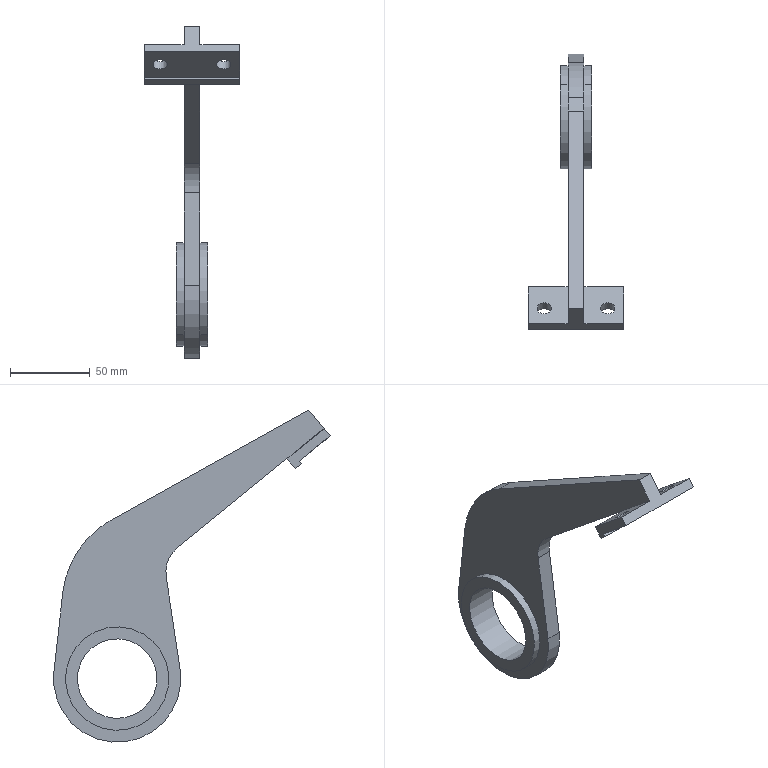Component | SolidWorks | OT-0100-003(SwingRod)-1 | 1 solid | 31 faces | box 60 x 173.77 x 208.81 mm | volume 126646 mm3 | plane 17 | cylinder 14 | commonest cylinder face diameters 9 x4 65 x4 50 x2 120 x2 40 x1 80 x1 | material Plain Carbon Steel
build123d program:
from build123d import *

# Parameters (mm, degrees)
BOSS_EXTRUDE1_DEPTH = 5
SKETCH2_R           = 32.5
BOSS_EXTRUDE2_DEPTH = 10
SKETCH3_R           = 25
CUT_EXTRUDE1_DEPTH  = 20
SKETCH4_W           = 60
SKETCH4_H           = 30
BOSS_EXTRUDE3_DEPTH = 8
CUT_EXTRUDE2_REACH  = 225.825
SKETCH5_W           = 2
SKETCH5_H           = 25
CUT_EXTRUDE3_REACH  = 219.486
SKETCH6_R           = 4.5


with BuildPart() as part:
    # Sketch1 → Boss-Extrude1 (new, symmetric)
    with BuildSketch(Plane(origin=(0, 0, 0), x_dir=(0, 0, -1), z_dir=(1, 0, 0))):
        with BuildLine():
            Line((-63.411, -7.471), (-28.535, 28.031))
            ThreePointArc((-28.535, 28.031), (31.516, 24.632), (20.308, -34.462))
            Line((20.308, -34.462), (-30.154, -64.198))
            ThreePointArc((-30.154, -64.198), (-37.365, -71.506), (-40, -81.429))
            Line((-40, -81.429), (-40, -200))
            Line((-40, -200), (-55, -200))
            Line((-55, -200), (-79.697, -59.937))
            ThreePointArc((-79.697, -59.937), (-77.911, -31.731), (-63.411, -7.471))
        make_face()
    extrude(amount=BOSS_EXTRUDE1_DEPTH, both=True)

    # Sketch2 → Boss-Extrude2 (add, symmetric)
    with BuildSketch(Plane(origin=(0, 0, 0), x_dir=(0, 0, -1), z_dir=(1, 0, 0))):
        with Locations(Location((0, 0, 0), (0, 0, 180))):
            Circle(SKETCH2_R)
    extrude(amount=BOSS_EXTRUDE2_DEPTH, both=True)

    # Sketch3 → Cut-Extrude1 (cut)
    with BuildSketch(Plane(origin=(10, 0, 0), x_dir=(0, 0, -1), z_dir=(1, 0, 0))):
        Circle(SKETCH3_R)
    extrude(amount=-CUT_EXTRUDE1_DEPTH, mode=Mode.SUBTRACT)

    # Sketch4 → Boss-Extrude3 (add)
    with BuildSketch(Plane(origin=(0, 0, 40), x_dir=(-1, 0, 0), z_dir=(0, 0, -1))):
        with Locations((0, -185)):
            Rectangle(SKETCH4_W, SKETCH4_H)
    extrude(amount=BOSS_EXTRUDE3_DEPTH)

    # Sketch5 → Cut-Extrude2 (cut, up to next)
    with BuildSketch(Plane(origin=(30, 0, 0), x_dir=(0, 0, -1), z_dir=(1, 0, 0)), mode=Mode.PRIVATE) as cut_extrude2_sk1:
        with Locations((-33, -187.5)):
            Rectangle(SKETCH5_W, SKETCH5_H)
    cut_extrude2_tool1 = extrude(cut_extrude2_sk1.sketch, amount=-CUT_EXTRUDE2_REACH, mode=Mode.PRIVATE) & part.part
    add(cut_extrude2_tool1.solids().sort_by_distance((30, -187.5, 33))[0], mode=Mode.SUBTRACT)

    # Sketch6 → Cut-Extrude3 (cut, up to next)
    with BuildSketch(Plane.XY.offset(40), mode=Mode.PRIVATE) as cut_extrude3_sk1:
        with Locations((20, -187.5)):
            Circle(SKETCH6_R)
    cut_extrude3_tool1 = extrude(cut_extrude3_sk1.sketch, amount=-CUT_EXTRUDE3_REACH, mode=Mode.PRIVATE) & part.part
    # Sketch6 → Cut-Extrude3 (cut, up to next)
    with BuildSketch(Plane.XY.offset(40), mode=Mode.PRIVATE) as cut_extrude3_sk2:
        with Locations((-20, -187.5)):
            Circle(SKETCH6_R)
    cut_extrude3_tool2 = extrude(cut_extrude3_sk2.sketch, amount=-CUT_EXTRUDE3_REACH, mode=Mode.PRIVATE) & part.part
    add(cut_extrude3_tool1.solids().sort_by_distance((20, -187.5, 40))[0], mode=Mode.SUBTRACT)
    add(cut_extrude3_tool2.solids().sort_by_distance((-20, -187.5, 40))[0], mode=Mode.SUBTRACT)


solid = part.part

# Placed as in the assembly
solid = solid.moved(Location((-20, 35, 0), (-39.097, 0, 0)))
STEP:
#1=COLOUR_RGB('',0.7922,0.8196,0.9333);
#2=FILL_AREA_STYLE_COLOUR('',#1);
#3=FILL_AREA_STYLE('',(#2));
#4=SURFACE_STYLE_FILL_AREA(#3);
#5=SURFACE_SIDE_STYLE('',(#4));
#6=SURFACE_STYLE_USAGE(.BOTH.,#5);
#7=PRESENTATION_STYLE_ASSIGNMENT((#6));
#8=CARTESIAN_POINT('',(-1.398,-3.507,5.694));
#9=VERTEX_POINT('',#8);
#10=CARTESIAN_POINT('',(-1.752,-3.507,5.694));
#11=VERTEX_POINT('',#10);
#12=CARTESIAN_POINT('',(-1.575,-3.507,5.694));
#13=DIRECTION('',(0.,-0.6306,-0.7761));
#14=DIRECTION('',(1.,0.,0.));
#15=AXIS2_PLACEMENT_3D('',#12,#13,#14);
#16=CIRCLE('',#15,0.1772);
#17=EDGE_CURVE('',#9,#11,#16,.T.);
#18=ORIENTED_EDGE('',*,*,#17,.T.);
#19=CARTESIAN_POINT('',(-1.752,-3.358,5.877));
#20=VERTEX_POINT('',#19);
#21=CARTESIAN_POINT('',(-1.752,-5.344,3.433));
#22=DIRECTION('',(-0.,0.6306,0.7761));
#23=VECTOR('',#22,39.37);
#24=LINE('',#21,#23);
#25=EDGE_CURVE('',#11,#20,#24,.T.);
#26=ORIENTED_EDGE('',*,*,#25,.T.);
#27=CARTESIAN_POINT('',(-1.398,-3.358,5.877));
#28=VERTEX_POINT('',#27);
#29=CARTESIAN_POINT('',(-1.575,-3.358,5.877));
#30=DIRECTION('',(-0.,0.6306,0.7761));
#31=DIRECTION('',(-1.,0.,0.));
#32=AXIS2_PLACEMENT_3D('',#29,#30,#31);
#33=CIRCLE('',#32,0.1772);
#34=EDGE_CURVE('',#20,#28,#33,.T.);
#35=ORIENTED_EDGE('',*,*,#34,.T.);
#36=CARTESIAN_POINT('',(-1.398,-5.344,3.433));
#37=DIRECTION('',(-0.,0.6306,0.7761));
#38=VECTOR('',#37,39.37);
#39=LINE('',#36,#38);
#40=EDGE_CURVE('',#9,#28,#39,.T.);
#41=ORIENTED_EDGE('',*,*,#40,.F.);
#42=EDGE_LOOP('',(#18,#26,#35,#41));
#43=FACE_OUTER_BOUND('',#42,.T.);
#44=CARTESIAN_POINT('',(-1.575,-5.344,3.433));
#45=DIRECTION('',(-0.,0.6306,0.7761));
#46=DIRECTION('',(1.,0.,0.));
#47=AXIS2_PLACEMENT_3D('',#44,#45,#46);
#48=CYLINDRICAL_SURFACE('',#47,0.1772);
#49=ADVANCED_FACE('',(#43),#48,.F.);
#50=CARTESIAN_POINT('',(0.1772,-3.507,5.694));
#51=VERTEX_POINT('',#50);
#52=CARTESIAN_POINT('',(-0.1772,-3.507,5.694));
#53=VERTEX_POINT('',#52);
#54=CARTESIAN_POINT('',(0.,-3.507,5.694));
#55=DIRECTION('',(0.,-0.6306,-0.7761));
#56=DIRECTION('',(1.,0.,0.));
#57=AXIS2_PLACEMENT_3D('',#54,#55,#56);
#58=CIRCLE('',#57,0.1772);
#59=EDGE_CURVE('',#51,#53,#58,.T.);
#60=ORIENTED_EDGE('',*,*,#59,.T.);
#61=CARTESIAN_POINT('',(-0.1772,-3.358,5.877));
#62=VERTEX_POINT('',#61);
#63=CARTESIAN_POINT('',(-0.1772,-5.344,3.433));
#64=DIRECTION('',(-0.,0.6306,0.7761));
#65=VECTOR('',#64,39.37);
#66=LINE('',#63,#65);
#67=EDGE_CURVE('',#53,#62,#66,.T.);
#68=ORIENTED_EDGE('',*,*,#67,.T.);
#69=CARTESIAN_POINT('',(0.1772,-3.358,5.877));
#70=VERTEX_POINT('',#69);
#71=CARTESIAN_POINT('',(0.,-3.358,5.877));
#72=DIRECTION('',(-0.,0.6306,0.7761));
#73=DIRECTION('',(1.,0.,0.));
#74=AXIS2_PLACEMENT_3D('',#71,#72,#73);
#75=CIRCLE('',#74,0.1772);
#76=EDGE_CURVE('',#62,#70,#75,.T.);
#77=ORIENTED_EDGE('',*,*,#76,.T.);
#78=CARTESIAN_POINT('',(0.1772,-5.344,3.433));
#79=DIRECTION('',(-0.,0.6306,0.7761));
#80=VECTOR('',#79,39.37);
#81=LINE('',#78,#80);
#82=EDGE_CURVE('',#51,#70,#81,.T.);
#83=ORIENTED_EDGE('',*,*,#82,.F.);
#84=EDGE_LOOP('',(#60,#68,#77,#83));
#85=FACE_OUTER_BOUND('',#84,.T.);
#86=CARTESIAN_POINT('',(0.,-5.344,3.433));
#87=DIRECTION('',(-0.,0.6306,0.7761));
#88=DIRECTION('',(1.,0.,0.));
#89=AXIS2_PLACEMENT_3D('',#86,#87,#88);
#90=CYLINDRICAL_SURFACE('',#89,0.1772);
#91=ADVANCED_FACE('',(#85),#90,.F.);
#92=CARTESIAN_POINT('',(-1.181,1.999,0.7639));
#93=VERTEX_POINT('',#92);
#94=CARTESIAN_POINT('',(-1.181,0.7573,-0.7639));
#95=VERTEX_POINT('',#94);
#96=CARTESIAN_POINT('',(-1.181,1.378,0.));
#97=DIRECTION('',(1.,0.,-0.));
#98=DIRECTION('',(0.,-0.6306,-0.7761));
#99=AXIS2_PLACEMENT_3D('',#96,#97,#98);
#100=CIRCLE('',#99,0.9843);
#101=EDGE_CURVE('',#93,#95,#100,.T.);
#102=ORIENTED_EDGE('',*,*,#101,.F.);
#103=CARTESIAN_POINT('',(-0.3937,1.999,0.7639));
#104=VERTEX_POINT('',#103);
#105=CARTESIAN_POINT('',(-1.181,1.999,0.7639));
#106=DIRECTION('',(1.,0.,-0.));
#107=VECTOR('',#106,39.37);
#108=LINE('',#105,#107);
#109=EDGE_CURVE('',#93,#104,#108,.T.);
#110=ORIENTED_EDGE('',*,*,#109,.T.);
#111=CARTESIAN_POINT('',(-0.3937,0.7573,-0.7639));
#112=VERTEX_POINT('',#111);
#113=CARTESIAN_POINT('',(-0.3937,1.378,0.));
#114=DIRECTION('',(1.,0.,-0.));
#115=DIRECTION('',(0.,-0.6306,-0.7761));
#116=AXIS2_PLACEMENT_3D('',#113,#114,#115);
#117=CIRCLE('',#116,0.9843);
#118=EDGE_CURVE('',#104,#112,#117,.T.);
#119=ORIENTED_EDGE('',*,*,#118,.T.);
#120=CARTESIAN_POINT('',(-1.181,0.7573,-0.7639));
#121=DIRECTION('',(1.,0.,-0.));
#122=VECTOR('',#121,39.37);
#123=LINE('',#120,#122);
#124=EDGE_CURVE('',#95,#112,#123,.T.);
#125=ORIENTED_EDGE('',*,*,#124,.F.);
#126=EDGE_LOOP('',(#102,#110,#119,#125));
#127=FACE_OUTER_BOUND('',#126,.T.);
#128=CARTESIAN_POINT('',(-1.181,1.378,0.));
#129=DIRECTION('',(1.,0.,-0.));
#130=DIRECTION('',(0.,-0.6306,-0.7761));
#131=AXIS2_PLACEMENT_3D('',#128,#129,#130);
#132=CYLINDRICAL_SURFACE('',#131,0.9843);
#133=ADVANCED_FACE('',(#127),#132,.F.);
#134=CARTESIAN_POINT('',(-0.3937,0.571,-0.993));
#135=VERTEX_POINT('',#134);
#136=CARTESIAN_POINT('',(-0.3937,2.185,0.993));
#137=VERTEX_POINT('',#136);
#138=CARTESIAN_POINT('',(-0.3937,1.378,0.));
#139=DIRECTION('',(1.,0.,-0.));
#140=DIRECTION('',(0.,-0.6306,-0.7761));
#141=AXIS2_PLACEMENT_3D('',#138,#139,#140);
#142=CIRCLE('',#141,1.28);
#143=EDGE_CURVE('',#135,#137,#142,.T.);
#144=ORIENTED_EDGE('',*,*,#143,.F.);
#145=CARTESIAN_POINT('',(-0.5906,0.571,-0.993));
#146=VERTEX_POINT('',#145);
#147=CARTESIAN_POINT('',(-0.3937,0.571,-0.993));
#148=DIRECTION('',(-1.,-0.,0.));
#149=VECTOR('',#148,39.37);
#150=LINE('',#147,#149);
#151=EDGE_CURVE('',#135,#146,#150,.T.);
#152=ORIENTED_EDGE('',*,*,#151,.T.);
#153=CARTESIAN_POINT('',(-0.5906,2.185,0.993));
#154=VERTEX_POINT('',#153);
#155=CARTESIAN_POINT('',(-0.5906,1.378,0.));
#156=DIRECTION('',(1.,0.,-0.));
#157=DIRECTION('',(0.,0.6306,0.7761));
#158=AXIS2_PLACEMENT_3D('',#155,#156,#157);
#159=CIRCLE('',#158,1.28);
#160=EDGE_CURVE('',#146,#154,#159,.T.);
#161=ORIENTED_EDGE('',*,*,#160,.T.);
#162=CARTESIAN_POINT('',(-0.3937,2.185,0.993));
#163=DIRECTION('',(-1.,-0.,0.));
#164=VECTOR('',#163,39.37);
#165=LINE('',#162,#164);
#166=EDGE_CURVE('',#137,#154,#165,.T.);
#167=ORIENTED_EDGE('',*,*,#166,.F.);
#168=EDGE_LOOP('',(#144,#152,#161,#167));
#169=FACE_OUTER_BOUND('',#168,.T.);
#170=CARTESIAN_POINT('',(-0.3937,1.378,0.));
#171=DIRECTION('',(-1.,-0.,0.));
#172=DIRECTION('',(0.,0.6306,0.7761));
#173=AXIS2_PLACEMENT_3D('',#170,#171,#172);
#174=CYLINDRICAL_SURFACE('',#173,1.28);
#175=ADVANCED_FACE('',(#169),#174,.T.);
#176=CARTESIAN_POINT('',(-0.9843,0.571,-0.993));
#177=VERTEX_POINT('',#176);
#178=CARTESIAN_POINT('',(-0.9843,2.185,0.993));
#179=VERTEX_POINT('',#178);
#180=CARTESIAN_POINT('',(-0.9843,1.378,0.));
#181=DIRECTION('',(1.,0.,-0.));
#182=DIRECTION('',(0.,0.6306,0.7761));
#183=AXIS2_PLACEMENT_3D('',#180,#181,#182);
#184=CIRCLE('',#183,1.28);
#185=EDGE_CURVE('',#177,#179,#184,.T.);
#186=ORIENTED_EDGE('',*,*,#185,.F.);
#187=CARTESIAN_POINT('',(-1.181,0.571,-0.993));
#188=VERTEX_POINT('',#187);
#189=CARTESIAN_POINT('',(-0.3937,0.571,-0.993));
#190=DIRECTION('',(-1.,-0.,0.));
#191=VECTOR('',#190,39.37);
#192=LINE('',#189,#191);
#193=EDGE_CURVE('',#177,#188,#192,.T.);
#194=ORIENTED_EDGE('',*,*,#193,.T.);
#195=CARTESIAN_POINT('',(-1.181,2.185,0.993));
#196=VERTEX_POINT('',#195);
#197=CARTESIAN_POINT('',(-1.181,1.378,0.));
#198=DIRECTION('',(1.,0.,-0.));
#199=DIRECTION('',(0.,-0.6306,-0.7761));
#200=AXIS2_PLACEMENT_3D('',#197,#198,#199);
#201=CIRCLE('',#200,1.28);
#202=EDGE_CURVE('',#188,#196,#201,.T.);
#203=ORIENTED_EDGE('',*,*,#202,.T.);
#204=CARTESIAN_POINT('',(-0.3937,2.185,0.993));
#205=DIRECTION('',(-1.,-0.,0.));
#206=VECTOR('',#205,39.37);
#207=LINE('',#204,#206);
#208=EDGE_CURVE('',#179,#196,#207,.T.);
#209=ORIENTED_EDGE('',*,*,#208,.F.);
#210=EDGE_LOOP('',(#186,#194,#203,#209));
#211=FACE_OUTER_BOUND('',#210,.T.);
#212=CARTESIAN_POINT('',(-0.3937,1.378,0.));
#213=DIRECTION('',(-1.,-0.,0.));
#214=DIRECTION('',(0.,0.6306,0.7761));
#215=AXIS2_PLACEMENT_3D('',#212,#213,#214);
#216=CYLINDRICAL_SURFACE('',#215,1.28);
#217=ADVANCED_FACE('',(#211),#216,.T.);
#218=CARTESIAN_POINT('',(-0.5906,1.866,3.692));
#219=VERTEX_POINT('',#218);
#220=CARTESIAN_POINT('',(-0.5906,1.525,3.923));
#221=VERTEX_POINT('',#220);
#222=CARTESIAN_POINT('',(-0.5906,0.3766,1.859));
#223=DIRECTION('',(1.,0.,-0.));
#224=DIRECTION('',(0.,-0.6306,-0.7761));
#225=AXIS2_PLACEMENT_3D('',#222,#223,#224);
#226=CIRCLE('',#225,2.362);
#227=EDGE_CURVE('',#219,#221,#226,.T.);
#228=ORIENTED_EDGE('',*,*,#227,.F.);
#229=CARTESIAN_POINT('',(-0.9843,1.866,3.692));
#230=VERTEX_POINT('',#229);
#231=CARTESIAN_POINT('',(-0.5906,1.866,3.692));
#232=DIRECTION('',(-1.,-0.,0.));
#233=VECTOR('',#232,39.37);
#234=LINE('',#231,#233);
#235=EDGE_CURVE('',#219,#230,#234,.T.);
#236=ORIENTED_EDGE('',*,*,#235,.T.);
#237=CARTESIAN_POINT('',(-0.9843,1.525,3.923));
#238=VERTEX_POINT('',#237);
#239=CARTESIAN_POINT('',(-0.9843,0.3766,1.859));
#240=DIRECTION('',(1.,0.,-0.));
#241=DIRECTION('',(0.,-0.6306,-0.7761));
#242=AXIS2_PLACEMENT_3D('',#239,#240,#241);
#243=CIRCLE('',#242,2.362);
#244=EDGE_CURVE('',#230,#238,#243,.T.);
#245=ORIENTED_EDGE('',*,*,#244,.T.);
#246=CARTESIAN_POINT('',(-0.5906,1.525,3.923));
#247=DIRECTION('',(-1.,-0.,0.));
#248=VECTOR('',#247,39.37);
#249=LINE('',#246,#248);
#250=EDGE_CURVE('',#221,#238,#249,.T.);
#251=ORIENTED_EDGE('',*,*,#250,.F.);
#252=EDGE_LOOP('',(#228,#236,#245,#251));
#253=FACE_OUTER_BOUND('',#252,.T.);
#254=CARTESIAN_POINT('',(-0.5906,0.3766,1.859));
#255=DIRECTION('',(-1.,-0.,0.));
#256=DIRECTION('',(0.,0.6306,0.7761));
#257=AXIS2_PLACEMENT_3D('',#254,#255,#256);
#258=CYLINDRICAL_SURFACE('',#257,2.362);
#259=ADVANCED_FACE('',(#253),#258,.T.);
#260=CARTESIAN_POINT('',(-0.9843,-2.823,5.443));
#261=VERTEX_POINT('',#260);
#262=CARTESIAN_POINT('',(-0.5906,-2.823,5.443));
#263=VERTEX_POINT('',#262);
#264=CARTESIAN_POINT('',(-0.5906,-2.823,5.443));
#265=DIRECTION('',(1.,0.,-0.));
#266=VECTOR('',#265,39.37);
#267=LINE('',#264,#266);
#268=EDGE_CURVE('',#261,#263,#267,.T.);
#269=ORIENTED_EDGE('',*,*,#268,.F.);
#270=CARTESIAN_POINT('',(-0.9843,-0.1169,3.244));
#271=VERTEX_POINT('',#270);
#272=CARTESIAN_POINT('',(-0.9843,-3.74,6.188));
#273=DIRECTION('',(-0.,0.7761,-0.6306));
#274=VECTOR('',#273,39.37);
#275=LINE('',#272,#274);
#276=EDGE_CURVE('',#261,#271,#275,.T.);
#277=ORIENTED_EDGE('',*,*,#276,.T.);
#278=CARTESIAN_POINT('',(-0.5906,-0.1169,3.244));
#279=VERTEX_POINT('',#278);
#280=CARTESIAN_POINT('',(-0.5906,-0.1169,3.244));
#281=DIRECTION('',(-1.,-0.,0.));
#282=VECTOR('',#281,39.37);
#283=LINE('',#280,#282);
#284=EDGE_CURVE('',#279,#271,#283,.T.);
#285=ORIENTED_EDGE('',*,*,#284,.F.);
#286=CARTESIAN_POINT('',(-0.5906,-3.74,6.188));
#287=DIRECTION('',(-0.,0.7761,-0.6306));
#288=VECTOR('',#287,39.37);
#289=LINE('',#286,#288);
#290=EDGE_CURVE('',#263,#279,#289,.T.);
#291=ORIENTED_EDGE('',*,*,#290,.F.);
#292=EDGE_LOOP('',(#269,#277,#285,#291));
#293=FACE_OUTER_BOUND('',#292,.T.);
#294=CARTESIAN_POINT('',(-0.5906,-3.74,6.188));
#295=DIRECTION('',(-0.,0.6306,0.7761));
#296=DIRECTION('',(0.,-0.7761,0.6306));
#297=AXIS2_PLACEMENT_3D('',#294,#295,#296);
#298=PLANE('',#297);
#299=ADVANCED_FACE('',(#293),#298,.F.);
#300=CARTESIAN_POINT('',(-0.5906,0.1651,2.515));
#301=VERTEX_POINT('',#300);
#302=CARTESIAN_POINT('',(-0.5906,-0.6135,2.633));
#303=DIRECTION('',(-1.,-0.,0.));
#304=DIRECTION('',(0.,0.6306,0.7761));
#305=AXIS2_PLACEMENT_3D('',#302,#303,#304);
#306=CIRCLE('',#305,0.7874);
#307=EDGE_CURVE('',#279,#301,#306,.T.);
#308=ORIENTED_EDGE('',*,*,#307,.T.);
#309=CARTESIAN_POINT('',(-0.5906,-0.1792,0.2351));
#310=VERTEX_POINT('',#309);
#311=CARTESIAN_POINT('',(-0.5906,0.1651,2.515));
#312=DIRECTION('',(-0.,-0.1493,-0.9888));
#313=VECTOR('',#312,39.37);
#314=LINE('',#311,#313);
#315=EDGE_CURVE('',#301,#310,#314,.T.);
#316=ORIENTED_EDGE('',*,*,#315,.T.);
#317=CARTESIAN_POINT('',(-0.5906,2.943,0.1759));
#318=VERTEX_POINT('',#317);
#319=CARTESIAN_POINT('',(-0.5906,1.378,0.));
#320=DIRECTION('',(1.,0.,-0.));
#321=DIRECTION('',(0.,-0.6306,-0.7761));
#322=AXIS2_PLACEMENT_3D('',#319,#320,#321);
#323=CIRCLE('',#322,1.575);
#324=EDGE_CURVE('',#310,#318,#323,.T.);
#325=ORIENTED_EDGE('',*,*,#324,.T.);
#326=CARTESIAN_POINT('',(-0.5906,2.724,2.123));
#327=VERTEX_POINT('',#326);
#328=CARTESIAN_POINT('',(-0.5906,2.724,2.123));
#329=DIRECTION('',(0.,-0.1117,0.9937));
#330=VECTOR('',#329,39.37);
#331=LINE('',#328,#330);
#332=EDGE_CURVE('',#318,#327,#331,.T.);
#333=ORIENTED_EDGE('',*,*,#332,.T.);
#334=CARTESIAN_POINT('',(-0.5906,0.3766,1.859));
#335=DIRECTION('',(1.,0.,-0.));
#336=DIRECTION('',(0.,-0.6306,-0.7761));
#337=AXIS2_PLACEMENT_3D('',#334,#335,#336);
#338=CIRCLE('',#337,2.362);
#339=EDGE_CURVE('',#327,#219,#338,.T.);
#340=ORIENTED_EDGE('',*,*,#339,.T.);
#341=ORIENTED_EDGE('',*,*,#227,.T.);
#342=CARTESIAN_POINT('',(-0.5906,-3.367,6.646));
#343=VERTEX_POINT('',#342);
#344=CARTESIAN_POINT('',(-0.5906,-3.367,6.646));
#345=DIRECTION('',(0.,-0.8738,0.4863));
#346=VECTOR('',#345,39.37);
#347=LINE('',#344,#346);
#348=EDGE_CURVE('',#221,#343,#347,.T.);
#349=ORIENTED_EDGE('',*,*,#348,.T.);
#350=CARTESIAN_POINT('',(-0.5906,-3.74,6.188));
#351=VERTEX_POINT('',#350);
#352=CARTESIAN_POINT('',(-0.5906,-3.367,6.646));
#353=DIRECTION('',(0.,-0.6306,-0.7761));
#354=VECTOR('',#353,39.37);
#355=LINE('',#352,#354);
#356=EDGE_CURVE('',#343,#351,#355,.T.);
#357=ORIENTED_EDGE('',*,*,#356,.T.);
#358=CARTESIAN_POINT('',(-0.5906,-3.74,6.188));
#359=DIRECTION('',(-0.,0.7761,-0.6306));
#360=VECTOR('',#359,39.37);
#361=LINE('',#358,#360);
#362=EDGE_CURVE('',#351,#263,#361,.T.);
#363=ORIENTED_EDGE('',*,*,#362,.T.);
#364=ORIENTED_EDGE('',*,*,#290,.T.);
#365=EDGE_LOOP('',(#308,#316,#325,#333,#340,#341,#349,#357,#363,#364));
#366=FACE_OUTER_BOUND('',#365,.T.);
#367=CARTESIAN_POINT('',(-0.5906,1.378,0.));
#368=DIRECTION('',(1.,0.,-0.));
#369=DIRECTION('',(0.,0.6306,0.7761));
#370=AXIS2_PLACEMENT_3D('',#367,#368,#369);
#371=CIRCLE('',#370,1.28);
#372=EDGE_CURVE('',#154,#146,#371,.T.);
#373=ORIENTED_EDGE('',*,*,#372,.F.);
#374=ORIENTED_EDGE('',*,*,#160,.F.);
#375=EDGE_LOOP('',(#373,#374));
#376=FACE_BOUND('',#375,.T.);
#377=CARTESIAN_POINT('',(-0.5906,-0.6135,2.633));
#378=DIRECTION('',(-1.,-0.,0.));
#379=DIRECTION('',(-0.,0.6306,0.7761));
#380=AXIS2_PLACEMENT_3D('',#377,#378,#379);
#381=PLANE('',#380);
#382=ADVANCED_FACE('',(#366,#376),#381,.F.);
#383=CARTESIAN_POINT('',(-0.9843,0.1651,2.515));
#384=VERTEX_POINT('',#383);
#385=CARTESIAN_POINT('',(-0.9843,-0.6135,2.633));
#386=DIRECTION('',(-1.,-0.,0.));
#387=DIRECTION('',(0.,0.6306,0.7761));
#388=AXIS2_PLACEMENT_3D('',#385,#386,#387);
#389=CIRCLE('',#388,0.7874);
#390=EDGE_CURVE('',#271,#384,#389,.T.);
#391=ORIENTED_EDGE('',*,*,#390,.F.);
#392=ORIENTED_EDGE('',*,*,#276,.F.);
#393=CARTESIAN_POINT('',(-0.9843,-3.74,6.188));
#394=VERTEX_POINT('',#393);
#395=CARTESIAN_POINT('',(-0.9843,-3.74,6.188));
#396=DIRECTION('',(-0.,0.7761,-0.6306));
#397=VECTOR('',#396,39.37);
#398=LINE('',#395,#397);
#399=EDGE_CURVE('',#394,#261,#398,.T.);
#400=ORIENTED_EDGE('',*,*,#399,.F.);
#401=CARTESIAN_POINT('',(-0.9843,-3.367,6.646));
#402=VERTEX_POINT('',#401);
#403=CARTESIAN_POINT('',(-0.9843,-3.367,6.646));
#404=DIRECTION('',(0.,-0.6306,-0.7761));
#405=VECTOR('',#404,39.37);
#406=LINE('',#403,#405);
#407=EDGE_CURVE('',#402,#394,#406,.T.);
#408=ORIENTED_EDGE('',*,*,#407,.F.);
#409=CARTESIAN_POINT('',(-0.9843,-3.367,6.646));
#410=DIRECTION('',(0.,-0.8738,0.4863));
#411=VECTOR('',#410,39.37);
#412=LINE('',#409,#411);
#413=EDGE_CURVE('',#238,#402,#412,.T.);
#414=ORIENTED_EDGE('',*,*,#413,.F.);
#415=ORIENTED_EDGE('',*,*,#244,.F.);
#416=CARTESIAN_POINT('',(-0.9843,2.724,2.123));
#417=VERTEX_POINT('',#416);
#418=CARTESIAN_POINT('',(-0.9843,0.3766,1.859));
#419=DIRECTION('',(1.,0.,-0.));
#420=DIRECTION('',(0.,-0.6306,-0.7761));
#421=AXIS2_PLACEMENT_3D('',#418,#419,#420);
#422=CIRCLE('',#421,2.362);
#423=EDGE_CURVE('',#417,#230,#422,.T.);
#424=ORIENTED_EDGE('',*,*,#423,.F.);
#425=CARTESIAN_POINT('',(-0.9843,2.943,0.1759));
#426=VERTEX_POINT('',#425);
#427=CARTESIAN_POINT('',(-0.9843,2.724,2.123));
#428=DIRECTION('',(0.,-0.1117,0.9937));
#429=VECTOR('',#428,39.37);
#430=LINE('',#427,#429);
#431=EDGE_CURVE('',#426,#417,#430,.T.);
#432=ORIENTED_EDGE('',*,*,#431,.F.);
#433=CARTESIAN_POINT('',(-0.9843,-0.1792,0.2351));
#434=VERTEX_POINT('',#433);
#435=CARTESIAN_POINT('',(-0.9843,1.378,0.));
#436=DIRECTION('',(1.,0.,-0.));
#437=DIRECTION('',(0.,-0.6306,-0.7761));
#438=AXIS2_PLACEMENT_3D('',#435,#436,#437);
#439=CIRCLE('',#438,1.575);
#440=EDGE_CURVE('',#434,#426,#439,.T.);
#441=ORIENTED_EDGE('',*,*,#440,.F.);
#442=CARTESIAN_POINT('',(-0.9843,0.1651,2.515));
#443=DIRECTION('',(-0.,-0.1493,-0.9888));
#444=VECTOR('',#443,39.37);
#445=LINE('',#442,#444);
#446=EDGE_CURVE('',#384,#434,#445,.T.);
#447=ORIENTED_EDGE('',*,*,#446,.F.);
#448=EDGE_LOOP('',(#391,#392,#400,#408,#414,#415,#424,#432,#441,#447));
#449=FACE_OUTER_BOUND('',#448,.T.);
#450=CARTESIAN_POINT('',(-0.9843,1.378,0.));
#451=DIRECTION('',(1.,0.,-0.));
#452=DIRECTION('',(0.,0.6306,0.7761));
#453=AXIS2_PLACEMENT_3D('',#450,#451,#452);
#454=CIRCLE('',#453,1.28);
#455=EDGE_CURVE('',#179,#177,#454,.T.);
#456=ORIENTED_EDGE('',*,*,#455,.T.);
#457=ORIENTED_EDGE('',*,*,#185,.T.);
#458=EDGE_LOOP('',(#456,#457));
#459=FACE_BOUND('',#458,.T.);
#460=CARTESIAN_POINT('',(-0.9843,-0.6135,2.633));
#461=DIRECTION('',(-1.,-0.,0.));
#462=DIRECTION('',(-0.,0.6306,0.7761));
#463=AXIS2_PLACEMENT_3D('',#460,#461,#462);
#464=PLANE('',#463);
#465=ADVANCED_FACE('',(#449,#459),#464,.T.);
#466=ORIENTED_EDGE('',*,*,#390,.T.);
#467=CARTESIAN_POINT('',(-0.5906,0.1651,2.515));
#468=DIRECTION('',(-1.,-0.,0.));
#469=VECTOR('',#468,39.37);
#470=LINE('',#467,#469);
#471=EDGE_CURVE('',#301,#384,#470,.T.);
#472=ORIENTED_EDGE('',*,*,#471,.F.);
#473=ORIENTED_EDGE('',*,*,#307,.F.);
#474=ORIENTED_EDGE('',*,*,#284,.T.);
#475=EDGE_LOOP('',(#466,#472,#473,#474));
#476=FACE_OUTER_BOUND('',#475,.T.);
#477=CARTESIAN_POINT('',(-0.5906,-0.6135,2.633));
#478=DIRECTION('',(-1.,-0.,0.));
#479=DIRECTION('',(0.,0.6306,0.7761));
#480=AXIS2_PLACEMENT_3D('',#477,#478,#479);
#481=CYLINDRICAL_SURFACE('',#480,0.7874);
#482=ADVANCED_FACE('',(#476),#481,.F.);
#483=ORIENTED_EDGE('',*,*,#446,.T.);
#484=CARTESIAN_POINT('',(-0.5906,-0.1792,0.2351));
#485=DIRECTION('',(-1.,-0.,0.));
#486=VECTOR('',#485,39.37);
#487=LINE('',#484,#486);
#488=EDGE_CURVE('',#310,#434,#487,.T.);
#489=ORIENTED_EDGE('',*,*,#488,.F.);
#490=ORIENTED_EDGE('',*,*,#315,.F.);
#491=ORIENTED_EDGE('',*,*,#471,.T.);
#492=EDGE_LOOP('',(#483,#489,#490,#491));
#493=FACE_OUTER_BOUND('',#492,.T.);
#494=CARTESIAN_POINT('',(-0.5906,0.1651,2.515));
#495=DIRECTION('',(-0.,0.9888,-0.1493));
#496=DIRECTION('',(0.,0.1493,0.9888));
#497=AXIS2_PLACEMENT_3D('',#494,#495,#496);
#498=PLANE('',#497);
#499=ADVANCED_FACE('',(#493),#498,.F.);
#500=ORIENTED_EDGE('',*,*,#440,.T.);
#501=CARTESIAN_POINT('',(-0.5906,2.943,0.1759));
#502=DIRECTION('',(-1.,-0.,0.));
#503=VECTOR('',#502,39.37);
#504=LINE('',#501,#503);
#505=EDGE_CURVE('',#318,#426,#504,.T.);
#506=ORIENTED_EDGE('',*,*,#505,.F.);
#507=ORIENTED_EDGE('',*,*,#324,.F.);
#508=ORIENTED_EDGE('',*,*,#488,.T.);
#509=EDGE_LOOP('',(#500,#506,#507,#508));
#510=FACE_OUTER_BOUND('',#509,.T.);
#511=CARTESIAN_POINT('',(-0.5906,1.378,0.));
#512=DIRECTION('',(-1.,-0.,0.));
#513=DIRECTION('',(0.,0.6306,0.7761));
#514=AXIS2_PLACEMENT_3D('',#511,#512,#513);
#515=CYLINDRICAL_SURFACE('',#514,1.575);
#516=ADVANCED_FACE('',(#510),#515,.T.);
#517=ORIENTED_EDGE('',*,*,#431,.T.);
#518=CARTESIAN_POINT('',(-0.5906,2.724,2.123));
#519=DIRECTION('',(-1.,-0.,0.));
#520=VECTOR('',#519,39.37);
#521=LINE('',#518,#520);
#522=EDGE_CURVE('',#327,#417,#521,.T.);
#523=ORIENTED_EDGE('',*,*,#522,.F.);
#524=ORIENTED_EDGE('',*,*,#332,.F.);
#525=ORIENTED_EDGE('',*,*,#505,.T.);
#526=EDGE_LOOP('',(#517,#523,#524,#525));
#527=FACE_OUTER_BOUND('',#526,.T.);
#528=CARTESIAN_POINT('',(-0.5906,2.724,2.123));
#529=DIRECTION('',(0.,-0.9937,-0.1117));
#530=DIRECTION('',(-0.,0.1117,-0.9937));
#531=AXIS2_PLACEMENT_3D('',#528,#529,#530);
#532=PLANE('',#531);
#533=ADVANCED_FACE('',(#527),#532,.F.);
#534=ORIENTED_EDGE('',*,*,#235,.F.);
#535=ORIENTED_EDGE('',*,*,#339,.F.);
#536=ORIENTED_EDGE('',*,*,#522,.T.);
#537=ORIENTED_EDGE('',*,*,#423,.T.);
#538=EDGE_LOOP('',(#534,#535,#536,#537));
#539=FACE_OUTER_BOUND('',#538,.T.);
#540=CARTESIAN_POINT('',(-0.5906,0.3766,1.859));
#541=DIRECTION('',(-1.,-0.,0.));
#542=DIRECTION('',(0.,0.6306,0.7761));
#543=AXIS2_PLACEMENT_3D('',#540,#541,#542);
#544=CYLINDRICAL_SURFACE('',#543,2.362);
#545=ADVANCED_FACE('',(#539),#544,.T.);
#546=ORIENTED_EDGE('',*,*,#413,.T.);
#547=CARTESIAN_POINT('',(-0.5906,-3.367,6.646));
#548=DIRECTION('',(-1.,-0.,0.));
#549=VECTOR('',#548,39.37);
#550=LINE('',#547,#549);
#551=EDGE_CURVE('',#343,#402,#550,.T.);
#552=ORIENTED_EDGE('',*,*,#551,.F.);
#553=ORIENTED_EDGE('',*,*,#348,.F.);
#554=ORIENTED_EDGE('',*,*,#250,.T.);
#555=EDGE_LOOP('',(#546,#552,#553,#554));
#556=FACE_OUTER_BOUND('',#555,.T.);
#557=CARTESIAN_POINT('',(-0.5906,-3.367,6.646));
#558=DIRECTION('',(-0.,-0.4863,-0.8738));
#559=DIRECTION('',(-0.,0.8738,-0.4863));
#560=AXIS2_PLACEMENT_3D('',#557,#558,#559);
#561=PLANE('',#560);
#562=ADVANCED_FACE('',(#556),#561,.F.);
#563=CARTESIAN_POINT('',(-1.969,-3.889,6.004));
#564=VERTEX_POINT('',#563);
#565=CARTESIAN_POINT('',(-1.969,-3.74,6.188));
#566=VERTEX_POINT('',#565);
#567=CARTESIAN_POINT('',(-1.969,-3.938,5.943));
#568=DIRECTION('',(-0.,0.6306,0.7761));
#569=VECTOR('',#568,39.37);
#570=LINE('',#567,#569);
#571=EDGE_CURVE('',#564,#566,#570,.T.);
#572=ORIENTED_EDGE('',*,*,#571,.F.);
#573=CARTESIAN_POINT('',(0.3937,-3.889,6.004));
#574=VERTEX_POINT('',#573);
#575=CARTESIAN_POINT('',(-1.969,-3.889,6.004));
#576=DIRECTION('',(1.,0.,-0.));
#577=VECTOR('',#576,39.37);
#578=LINE('',#575,#577);
#579=EDGE_CURVE('',#564,#574,#578,.T.);
#580=ORIENTED_EDGE('',*,*,#579,.T.);
#581=CARTESIAN_POINT('',(0.3937,-3.74,6.188));
#582=VERTEX_POINT('',#581);
#583=CARTESIAN_POINT('',(0.3937,-3.938,5.943));
#584=DIRECTION('',(-0.,0.6306,0.7761));
#585=VECTOR('',#584,39.37);
#586=LINE('',#583,#585);
#587=EDGE_CURVE('',#574,#582,#586,.T.);
#588=ORIENTED_EDGE('',*,*,#587,.T.);
#589=CARTESIAN_POINT('',(0.3937,-3.74,6.188));
#590=DIRECTION('',(-1.,-0.,0.));
#591=VECTOR('',#590,39.37);
#592=LINE('',#589,#591);
#593=EDGE_CURVE('',#582,#351,#592,.T.);
#594=ORIENTED_EDGE('',*,*,#593,.T.);
#595=ORIENTED_EDGE('',*,*,#356,.F.);
#596=ORIENTED_EDGE('',*,*,#551,.T.);
#597=ORIENTED_EDGE('',*,*,#407,.T.);
#598=CARTESIAN_POINT('',(0.3937,-3.74,6.188));
#599=DIRECTION('',(-1.,-0.,0.));
#600=VECTOR('',#599,39.37);
#601=LINE('',#598,#600);
#602=EDGE_CURVE('',#394,#566,#601,.T.);
#603=ORIENTED_EDGE('',*,*,#602,.T.);
#604=EDGE_LOOP('',(#572,#580,#588,#594,#595,#596,#597,#603));
#605=FACE_OUTER_BOUND('',#604,.T.);
#606=CARTESIAN_POINT('',(-0.5906,-3.367,6.646));
#607=DIRECTION('',(-0.,0.7761,-0.6306));
#608=DIRECTION('',(-0.,0.6306,0.7761));
#609=AXIS2_PLACEMENT_3D('',#606,#607,#608);
#610=PLANE('',#609);
#611=ADVANCED_FACE('',(#605),#610,.F.);
#612=CARTESIAN_POINT('',(-1.181,1.378,0.));
#613=DIRECTION('',(1.,0.,-0.));
#614=DIRECTION('',(0.,-0.6306,-0.7761));
#615=AXIS2_PLACEMENT_3D('',#612,#613,#614);
#616=CIRCLE('',#615,0.9843);
#617=EDGE_CURVE('',#95,#93,#616,.T.);
#618=ORIENTED_EDGE('',*,*,#617,.T.);
#619=ORIENTED_EDGE('',*,*,#101,.T.);
#620=EDGE_LOOP('',(#618,#619));
#621=FACE_BOUND('',#620,.T.);
#622=CARTESIAN_POINT('',(-1.181,1.378,0.));
#623=DIRECTION('',(1.,0.,-0.));
#624=DIRECTION('',(0.,-0.6306,-0.7761));
#625=AXIS2_PLACEMENT_3D('',#622,#623,#624);
#626=CIRCLE('',#625,1.28);
#627=EDGE_CURVE('',#196,#188,#626,.T.);
#628=ORIENTED_EDGE('',*,*,#627,.F.);
#629=ORIENTED_EDGE('',*,*,#202,.F.);
#630=EDGE_LOOP('',(#628,#629));
#631=FACE_OUTER_BOUND('',#630,.T.);
#632=CARTESIAN_POINT('',(-1.181,1.378,0.));
#633=DIRECTION('',(1.,0.,-0.));
#634=DIRECTION('',(0.,-0.6306,-0.7761));
#635=AXIS2_PLACEMENT_3D('',#632,#633,#634);
#636=PLANE('',#635);
#637=ADVANCED_FACE('',(#621,#631),#636,.F.);
#638=ORIENTED_EDGE('',*,*,#193,.F.);
#639=ORIENTED_EDGE('',*,*,#455,.F.);
#640=ORIENTED_EDGE('',*,*,#208,.T.);
#641=ORIENTED_EDGE('',*,*,#627,.T.);
#642=EDGE_LOOP('',(#638,#639,#640,#641));
#643=FACE_OUTER_BOUND('',#642,.T.);
#644=CARTESIAN_POINT('',(-0.3937,1.378,0.));
#645=DIRECTION('',(-1.,-0.,0.));
#646=DIRECTION('',(0.,0.6306,0.7761));
#647=AXIS2_PLACEMENT_3D('',#644,#645,#646);
#648=CYLINDRICAL_SURFACE('',#647,1.28);
#649=ADVANCED_FACE('',(#643),#648,.T.);
#650=ORIENTED_EDGE('',*,*,#151,.F.);
#651=CARTESIAN_POINT('',(-0.3937,1.378,0.));
#652=DIRECTION('',(1.,0.,-0.));
#653=DIRECTION('',(0.,-0.6306,-0.7761));
#654=AXIS2_PLACEMENT_3D('',#651,#652,#653);
#655=CIRCLE('',#654,1.28);
#656=EDGE_CURVE('',#137,#135,#655,.T.);
#657=ORIENTED_EDGE('',*,*,#656,.F.);
#658=ORIENTED_EDGE('',*,*,#166,.T.);
#659=ORIENTED_EDGE('',*,*,#372,.T.);
#660=EDGE_LOOP('',(#650,#657,#658,#659));
#661=FACE_OUTER_BOUND('',#660,.T.);
#662=CARTESIAN_POINT('',(-0.3937,1.378,0.));
#663=DIRECTION('',(-1.,-0.,0.));
#664=DIRECTION('',(0.,0.6306,0.7761));
#665=AXIS2_PLACEMENT_3D('',#662,#663,#664);
#666=CYLINDRICAL_SURFACE('',#665,1.28);
#667=ADVANCED_FACE('',(#661),#666,.T.);
#668=CARTESIAN_POINT('',(-0.3937,1.378,0.));
#669=DIRECTION('',(1.,0.,-0.));
#670=DIRECTION('',(0.,-0.6306,-0.7761));
#671=AXIS2_PLACEMENT_3D('',#668,#669,#670);
#672=CIRCLE('',#671,0.9843);
#673=EDGE_CURVE('',#112,#104,#672,.T.);
#674=ORIENTED_EDGE('',*,*,#673,.F.);
#675=ORIENTED_EDGE('',*,*,#118,.F.);
#676=EDGE_LOOP('',(#674,#675));
#677=FACE_BOUND('',#676,.T.);
#678=ORIENTED_EDGE('',*,*,#656,.T.);
#679=ORIENTED_EDGE('',*,*,#143,.T.);
#680=EDGE_LOOP('',(#678,#679));
#681=FACE_OUTER_BOUND('',#680,.T.);
#682=CARTESIAN_POINT('',(-0.3937,1.378,0.));
#683=DIRECTION('',(1.,0.,-0.));
#684=DIRECTION('',(0.,-0.6306,-0.7761));
#685=AXIS2_PLACEMENT_3D('',#682,#683,#684);
#686=PLANE('',#685);
#687=ADVANCED_FACE('',(#677,#681),#686,.T.);
#688=ORIENTED_EDGE('',*,*,#109,.F.);
#689=ORIENTED_EDGE('',*,*,#617,.F.);
#690=ORIENTED_EDGE('',*,*,#124,.T.);
#691=ORIENTED_EDGE('',*,*,#673,.T.);
#692=EDGE_LOOP('',(#688,#689,#690,#691));
#693=FACE_OUTER_BOUND('',#692,.T.);
#694=CARTESIAN_POINT('',(-1.181,1.378,0.));
#695=DIRECTION('',(1.,0.,-0.));
#696=DIRECTION('',(0.,-0.6306,-0.7761));
#697=AXIS2_PLACEMENT_3D('',#694,#695,#696);
#698=CYLINDRICAL_SURFACE('',#697,0.9843);
#699=ADVANCED_FACE('',(#693),#698,.F.);
#700=CARTESIAN_POINT('',(0.,-3.358,5.877));
#701=DIRECTION('',(-0.,0.6306,0.7761));
#702=DIRECTION('',(1.,0.,0.));
#703=AXIS2_PLACEMENT_3D('',#700,#701,#702);
#704=CIRCLE('',#703,0.1772);
#705=EDGE_CURVE('',#70,#62,#704,.T.);
#706=ORIENTED_EDGE('',*,*,#705,.F.);
#707=ORIENTED_EDGE('',*,*,#76,.F.);
#708=EDGE_LOOP('',(#706,#707));
#709=FACE_BOUND('',#708,.T.);
#710=ORIENTED_EDGE('',*,*,#362,.F.);
#711=ORIENTED_EDGE('',*,*,#593,.F.);
#712=CARTESIAN_POINT('',(0.3937,-2.823,5.443));
#713=VERTEX_POINT('',#712);
#714=CARTESIAN_POINT('',(0.3937,-3.74,6.188));
#715=DIRECTION('',(0.,-0.7761,0.6306));
#716=VECTOR('',#715,39.37);
#717=LINE('',#714,#716);
#718=EDGE_CURVE('',#713,#582,#717,.T.);
#719=ORIENTED_EDGE('',*,*,#718,.F.);
#720=CARTESIAN_POINT('',(0.3937,-2.823,5.443));
#721=DIRECTION('',(1.,0.,-0.));
#722=VECTOR('',#721,39.37);
#723=LINE('',#720,#722);
#724=EDGE_CURVE('',#263,#713,#723,.T.);
#725=ORIENTED_EDGE('',*,*,#724,.F.);
#726=EDGE_LOOP('',(#710,#711,#719,#725));
#727=FACE_OUTER_BOUND('',#726,.T.);
#728=CARTESIAN_POINT('',(-0.7874,2.371,1.222));
#729=DIRECTION('',(-0.,0.6306,0.7761));
#730=DIRECTION('',(0.,-0.7761,0.6306));
#731=AXIS2_PLACEMENT_3D('',#728,#729,#730);
#732=PLANE('',#731);
#733=ADVANCED_FACE('',(#709,#727),#732,.T.);
#734=CARTESIAN_POINT('',(-1.969,-3.125,5.384));
#735=VERTEX_POINT('',#734);
#736=CARTESIAN_POINT('',(-1.969,-3.175,5.323));
#737=VERTEX_POINT('',#736);
#738=CARTESIAN_POINT('',(-1.969,-3.175,5.323));
#739=DIRECTION('',(0.,-0.6306,-0.7761));
#740=VECTOR('',#739,39.37);
#741=LINE('',#738,#740);
#742=EDGE_CURVE('',#735,#737,#741,.T.);
#743=ORIENTED_EDGE('',*,*,#742,.F.);
#744=CARTESIAN_POINT('',(-1.969,-3.889,6.004));
#745=DIRECTION('',(-0.,0.7761,-0.6306));
#746=VECTOR('',#745,39.37);
#747=LINE('',#744,#746);
#748=EDGE_CURVE('',#564,#735,#747,.T.);
#749=ORIENTED_EDGE('',*,*,#748,.F.);
#750=ORIENTED_EDGE('',*,*,#571,.T.);
#751=CARTESIAN_POINT('',(-1.969,-2.823,5.443));
#752=VERTEX_POINT('',#751);
#753=CARTESIAN_POINT('',(-1.969,-3.74,6.188));
#754=DIRECTION('',(-0.,0.7761,-0.6306));
#755=VECTOR('',#754,39.37);
#756=LINE('',#753,#755);
#757=EDGE_CURVE('',#566,#752,#756,.T.);
#758=ORIENTED_EDGE('',*,*,#757,.T.);
#759=CARTESIAN_POINT('',(-1.969,-3.022,5.199));
#760=VERTEX_POINT('',#759);
#761=CARTESIAN_POINT('',(-1.969,-3.022,5.199));
#762=DIRECTION('',(-0.,0.6306,0.7761));
#763=VECTOR('',#762,39.37);
#764=LINE('',#761,#763);
#765=EDGE_CURVE('',#760,#752,#764,.T.);
#766=ORIENTED_EDGE('',*,*,#765,.F.);
#767=CARTESIAN_POINT('',(-1.969,-3.938,5.943));
#768=DIRECTION('',(-0.,0.7761,-0.6306));
#769=VECTOR('',#768,39.37);
#770=LINE('',#767,#769);
#771=EDGE_CURVE('',#737,#760,#770,.T.);
#772=ORIENTED_EDGE('',*,*,#771,.F.);
#773=EDGE_LOOP('',(#743,#749,#750,#758,#766,#772));
#774=FACE_OUTER_BOUND('',#773,.T.);
#775=CARTESIAN_POINT('',(-1.969,-3.938,5.943));
#776=DIRECTION('',(1.,0.,-0.));
#777=DIRECTION('',(0.,-0.6306,-0.7761));
#778=AXIS2_PLACEMENT_3D('',#775,#776,#777);
#779=PLANE('',#778);
#780=ADVANCED_FACE('',(#774),#779,.F.);
#781=CARTESIAN_POINT('',(0.3937,-2.823,5.443));
#782=DIRECTION('',(1.,0.,-0.));
#783=VECTOR('',#782,39.37);
#784=LINE('',#781,#783);
#785=EDGE_CURVE('',#752,#261,#784,.T.);
#786=ORIENTED_EDGE('',*,*,#785,.T.);
#787=ORIENTED_EDGE('',*,*,#268,.T.);
#788=ORIENTED_EDGE('',*,*,#724,.T.);
#789=CARTESIAN_POINT('',(0.3937,-3.022,5.199));
#790=VERTEX_POINT('',#789);
#791=CARTESIAN_POINT('',(0.3937,-3.022,5.199));
#792=DIRECTION('',(-0.,0.6306,0.7761));
#793=VECTOR('',#792,39.37);
#794=LINE('',#791,#793);
#795=EDGE_CURVE('',#790,#713,#794,.T.);
#796=ORIENTED_EDGE('',*,*,#795,.F.);
#797=CARTESIAN_POINT('',(0.3937,-3.022,5.199));
#798=DIRECTION('',(1.,0.,-0.));
#799=VECTOR('',#798,39.37);
#800=LINE('',#797,#799);
#801=EDGE_CURVE('',#760,#790,#800,.T.);
#802=ORIENTED_EDGE('',*,*,#801,.F.);
#803=ORIENTED_EDGE('',*,*,#765,.T.);
#804=EDGE_LOOP('',(#786,#787,#788,#796,#802,#803));
#805=FACE_OUTER_BOUND('',#804,.T.);
#806=CARTESIAN_POINT('',(0.3937,-3.022,5.199));
#807=DIRECTION('',(0.,-0.7761,0.6306));
#808=DIRECTION('',(0.,-0.6306,-0.7761));
#809=AXIS2_PLACEMENT_3D('',#806,#807,#808);
#810=PLANE('',#809);
#811=ADVANCED_FACE('',(#805),#810,.F.);
#812=ORIENTED_EDGE('',*,*,#587,.F.);
#813=CARTESIAN_POINT('',(0.3937,-3.125,5.384));
#814=VERTEX_POINT('',#813);
#815=CARTESIAN_POINT('',(0.3937,-3.889,6.004));
#816=DIRECTION('',(0.,-0.7761,0.6306));
#817=VECTOR('',#816,39.37);
#818=LINE('',#815,#817);
#819=EDGE_CURVE('',#814,#574,#818,.T.);
#820=ORIENTED_EDGE('',*,*,#819,.F.);
#821=CARTESIAN_POINT('',(0.3937,-3.175,5.323));
#822=VERTEX_POINT('',#821);
#823=CARTESIAN_POINT('',(0.3937,-3.175,5.323));
#824=DIRECTION('',(-0.,0.6306,0.7761));
#825=VECTOR('',#824,39.37);
#826=LINE('',#823,#825);
#827=EDGE_CURVE('',#822,#814,#826,.T.);
#828=ORIENTED_EDGE('',*,*,#827,.F.);
#829=CARTESIAN_POINT('',(0.3937,-3.938,5.943));
#830=DIRECTION('',(0.,-0.7761,0.6306));
#831=VECTOR('',#830,39.37);
#832=LINE('',#829,#831);
#833=EDGE_CURVE('',#790,#822,#832,.T.);
#834=ORIENTED_EDGE('',*,*,#833,.F.);
#835=ORIENTED_EDGE('',*,*,#795,.T.);
#836=ORIENTED_EDGE('',*,*,#718,.T.);
#837=EDGE_LOOP('',(#812,#820,#828,#834,#835,#836));
#838=FACE_OUTER_BOUND('',#837,.T.);
#839=CARTESIAN_POINT('',(0.3937,-3.938,5.943));
#840=DIRECTION('',(-1.,-0.,0.));
#841=DIRECTION('',(-0.,0.6306,0.7761));
#842=AXIS2_PLACEMENT_3D('',#839,#840,#841);
#843=PLANE('',#842);
#844=ADVANCED_FACE('',(#838),#843,.F.);
#845=ORIENTED_EDGE('',*,*,#833,.T.);
#846=CARTESIAN_POINT('',(-1.969,-3.175,5.323));
#847=DIRECTION('',(1.,0.,-0.));
#848=VECTOR('',#847,39.37);
#849=LINE('',#846,#848);
#850=EDGE_CURVE('',#737,#822,#849,.T.);
#851=ORIENTED_EDGE('',*,*,#850,.F.);
#852=ORIENTED_EDGE('',*,*,#771,.T.);
#853=ORIENTED_EDGE('',*,*,#801,.T.);
#854=EDGE_LOOP('',(#845,#851,#852,#853));
#855=FACE_OUTER_BOUND('',#854,.T.);
#856=CARTESIAN_POINT('',(-0.7874,2.172,0.9777));
#857=DIRECTION('',(-0.,0.6306,0.7761));
#858=DIRECTION('',(0.,-0.7761,0.6306));
#859=AXIS2_PLACEMENT_3D('',#856,#857,#858);
#860=PLANE('',#859);
#861=ADVANCED_FACE('',(#855),#860,.F.);
#862=CARTESIAN_POINT('',(-1.575,-3.358,5.877));
#863=DIRECTION('',(-0.,0.6306,0.7761));
#864=DIRECTION('',(-1.,0.,0.));
#865=AXIS2_PLACEMENT_3D('',#862,#863,#864);
#866=CIRCLE('',#865,0.1772);
#867=EDGE_CURVE('',#28,#20,#866,.T.);
#868=ORIENTED_EDGE('',*,*,#867,.F.);
#869=ORIENTED_EDGE('',*,*,#34,.F.);
#870=EDGE_LOOP('',(#868,#869));
#871=FACE_BOUND('',#870,.T.);
#872=ORIENTED_EDGE('',*,*,#602,.F.);
#873=ORIENTED_EDGE('',*,*,#399,.T.);
#874=ORIENTED_EDGE('',*,*,#785,.F.);
#875=ORIENTED_EDGE('',*,*,#757,.F.);
#876=EDGE_LOOP('',(#872,#873,#874,#875));
#877=FACE_OUTER_BOUND('',#876,.T.);
#878=CARTESIAN_POINT('',(-0.7874,2.371,1.222));
#879=DIRECTION('',(-0.,0.6306,0.7761));
#880=DIRECTION('',(0.,-0.7761,0.6306));
#881=AXIS2_PLACEMENT_3D('',#878,#879,#880);
#882=PLANE('',#881);
#883=ADVANCED_FACE('',(#871,#877),#882,.T.);
#884=ORIENTED_EDGE('',*,*,#17,.F.);
#885=CARTESIAN_POINT('',(-1.575,-3.507,5.694));
#886=DIRECTION('',(0.,-0.6306,-0.7761));
#887=DIRECTION('',(1.,-0.,0.));
#888=AXIS2_PLACEMENT_3D('',#885,#886,#887);
#889=CIRCLE('',#888,0.1772);
#890=EDGE_CURVE('',#11,#9,#889,.T.);
#891=ORIENTED_EDGE('',*,*,#890,.F.);
#892=EDGE_LOOP('',(#884,#891));
#893=FACE_BOUND('',#892,.T.);
#894=ORIENTED_EDGE('',*,*,#59,.F.);
#895=CARTESIAN_POINT('',(0.,-3.507,5.694));
#896=DIRECTION('',(0.,-0.6306,-0.7761));
#897=DIRECTION('',(1.,-0.,0.));
#898=AXIS2_PLACEMENT_3D('',#895,#896,#897);
#899=CIRCLE('',#898,0.1772);
#900=EDGE_CURVE('',#53,#51,#899,.T.);
#901=ORIENTED_EDGE('',*,*,#900,.F.);
#902=EDGE_LOOP('',(#894,#901));
#903=FACE_BOUND('',#902,.T.);
#904=ORIENTED_EDGE('',*,*,#748,.T.);
#905=CARTESIAN_POINT('',(-1.969,-3.125,5.384));
#906=DIRECTION('',(1.,0.,-0.));
#907=VECTOR('',#906,39.37);
#908=LINE('',#905,#907);
#909=EDGE_CURVE('',#735,#814,#908,.T.);
#910=ORIENTED_EDGE('',*,*,#909,.T.);
#911=ORIENTED_EDGE('',*,*,#819,.T.);
#912=ORIENTED_EDGE('',*,*,#579,.F.);
#913=EDGE_LOOP('',(#904,#910,#911,#912));
#914=FACE_OUTER_BOUND('',#913,.T.);
#915=CARTESIAN_POINT('',(-1.969,-3.889,6.004));
#916=DIRECTION('',(-0.,0.6306,0.7761));
#917=DIRECTION('',(1.,0.,-0.));
#918=AXIS2_PLACEMENT_3D('',#915,#916,#917);
#919=PLANE('',#918);
#920=ADVANCED_FACE('',(#893,#903,#914),#919,.F.);
#921=ORIENTED_EDGE('',*,*,#742,.T.);
#922=ORIENTED_EDGE('',*,*,#850,.T.);
#923=ORIENTED_EDGE('',*,*,#827,.T.);
#924=ORIENTED_EDGE('',*,*,#909,.F.);
#925=EDGE_LOOP('',(#921,#922,#923,#924));
#926=FACE_OUTER_BOUND('',#925,.T.);
#927=CARTESIAN_POINT('',(-1.969,-3.175,5.323));
#928=DIRECTION('',(-0.,0.7761,-0.6306));
#929=DIRECTION('',(-0.,0.6306,0.7761));
#930=AXIS2_PLACEMENT_3D('',#927,#928,#929);
#931=PLANE('',#930);
#932=ADVANCED_FACE('',(#926),#931,.F.);
#933=ORIENTED_EDGE('',*,*,#67,.F.);
#934=ORIENTED_EDGE('',*,*,#900,.T.);
#935=ORIENTED_EDGE('',*,*,#82,.T.);
#936=ORIENTED_EDGE('',*,*,#705,.T.);
#937=EDGE_LOOP('',(#933,#934,#935,#936));
#938=FACE_OUTER_BOUND('',#937,.T.);
#939=CARTESIAN_POINT('',(0.,-5.344,3.433));
#940=DIRECTION('',(-0.,0.6306,0.7761));
#941=DIRECTION('',(1.,0.,0.));
#942=AXIS2_PLACEMENT_3D('',#939,#940,#941);
#943=CYLINDRICAL_SURFACE('',#942,0.1772);
#944=ADVANCED_FACE('',(#938),#943,.F.);
#945=ORIENTED_EDGE('',*,*,#25,.F.);
#946=ORIENTED_EDGE('',*,*,#890,.T.);
#947=ORIENTED_EDGE('',*,*,#40,.T.);
#948=ORIENTED_EDGE('',*,*,#867,.T.);
#949=EDGE_LOOP('',(#945,#946,#947,#948));
#950=FACE_OUTER_BOUND('',#949,.T.);
#951=CARTESIAN_POINT('',(-1.575,-5.344,3.433));
#952=DIRECTION('',(-0.,0.6306,0.7761));
#953=DIRECTION('',(1.,0.,0.));
#954=AXIS2_PLACEMENT_3D('',#951,#952,#953);
#955=CYLINDRICAL_SURFACE('',#954,0.1772);
#956=ADVANCED_FACE('',(#950),#955,.F.);
#957=CLOSED_SHELL('',(#49,#91,#133,#175,#217,#259,#299,#382,#465,#482,#499,#516,#533,#545,#562,#611,#637,#649,#667,#687,#699,#733,#780,#811,#844,#861,#883,#920,#932,#944,#956));
#958=MANIFOLD_SOLID_BREP('',#957);
#959=STYLED_ITEM('',(#7),#958);
#960=(LENGTH_UNIT()NAMED_UNIT(*)SI_UNIT($,.METRE.));
#961=LENGTH_MEASURE_WITH_UNIT(LENGTH_MEASURE(0.0254),#960);
#962=DIMENSIONAL_EXPONENTS(1.,0.,0.,0.,0.,0.,0.);
#963=(CONVERSION_BASED_UNIT('',#961)LENGTH_UNIT()NAMED_UNIT(#962));
#964=UNCERTAINTY_MEASURE_WITH_UNIT(LENGTH_MEASURE(0.00001),#963,'','');
#965=(NAMED_UNIT(*)PLANE_ANGLE_UNIT()SI_UNIT($,.RADIAN.));
#966=(NAMED_UNIT(*)SI_UNIT($,.STERADIAN.)SOLID_ANGLE_UNIT());
#967=(GEOMETRIC_REPRESENTATION_CONTEXT(3)GLOBAL_UNCERTAINTY_ASSIGNED_CONTEXT((#964))GLOBAL_UNIT_ASSIGNED_CONTEXT((#963,#965,#966))REPRESENTATION_CONTEXT('',''));
#968=MECHANICAL_DESIGN_GEOMETRIC_PRESENTATION_REPRESENTATION('',(#959),#967);
#969=PRESENTATION_LAYER_ASSIGNMENT('','',(#959));
#970=CARTESIAN_POINT('',(0.,0.,0.));
#971=DIRECTION('',(0.,0.,1.));
#972=DIRECTION('',(1.,0.,0.));
#973=AXIS2_PLACEMENT_3D('',#970,#971,#972);
#974=(LENGTH_UNIT()NAMED_UNIT(*)SI_UNIT($,.METRE.));
#975=LENGTH_MEASURE_WITH_UNIT(LENGTH_MEASURE(0.0254),#974);
#976=DIMENSIONAL_EXPONENTS(1.,0.,0.,0.,0.,0.,0.);
#977=(CONVERSION_BASED_UNIT('',#975)LENGTH_UNIT()NAMED_UNIT(#976));
#978=UNCERTAINTY_MEASURE_WITH_UNIT(LENGTH_MEASURE(0.00001),#977,'','');
#979=(NAMED_UNIT(*)PLANE_ANGLE_UNIT()SI_UNIT($,.RADIAN.));
#980=(NAMED_UNIT(*)SI_UNIT($,.STERADIAN.)SOLID_ANGLE_UNIT());
#981=(GEOMETRIC_REPRESENTATION_CONTEXT(3)GLOBAL_UNCERTAINTY_ASSIGNED_CONTEXT((#978))GLOBAL_UNIT_ASSIGNED_CONTEXT((#977,#979,#980))REPRESENTATION_CONTEXT('',''));
#982=ADVANCED_BREP_SHAPE_REPRESENTATION('',(#958,#973),#981);